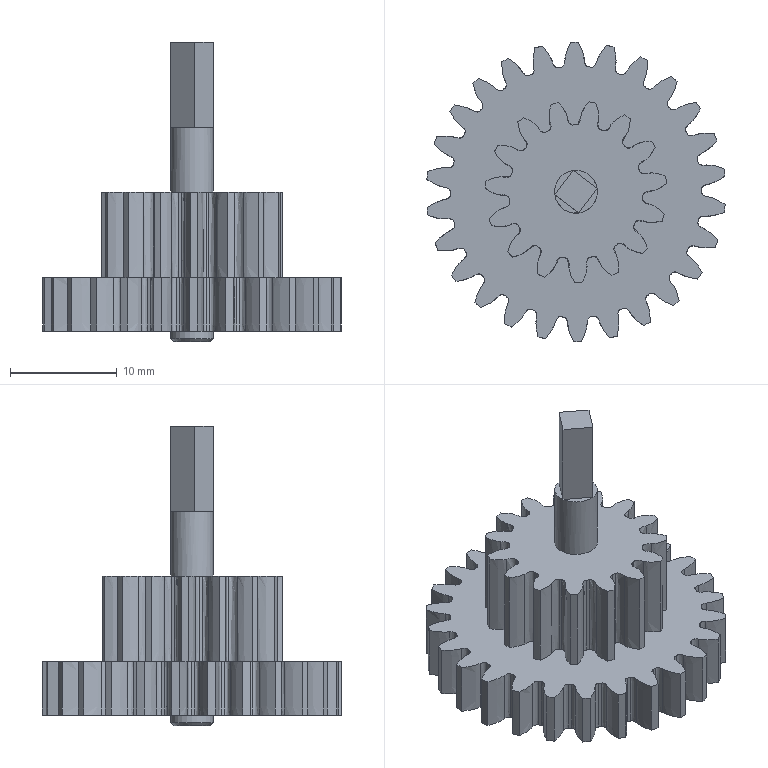Component | NX | GEAR_1 | 1 solid | 262 faces | volume 4151 mm3 | other 205 | cylinder 43 | plane 13 | cone 1 | commonest cylinder face diameters 23.5 x26 12.5 x15 4 x2